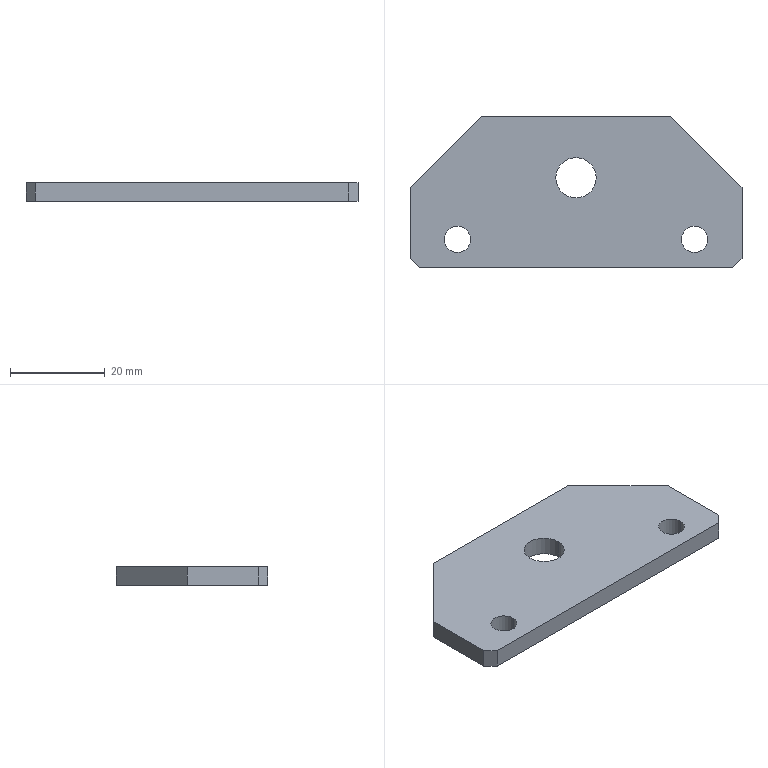Component | SolidWorks | DZ.KX.203-TC1505-30-09-01-05-03-4 | 1 solid | 16 faces | box 70 x 32 x 4 mm | volume 7627 mm3 | plane 10 | cylinder 6 | commonest cylinder face diameters 5.5 x4 8.5 x2
build123d program:
from build123d import *

# Parameters (mm, degrees)
SKETCH1_W                      = 70
SKETCH1_H                      = 32
BOSS_EXTRUDE1_DEPTH            = 4
HOLE1_D                        = 8.5
CHAMFER1_SIZE                  = 15
F_5_5_5_5_DIAMETER_HOLE1_D     = 5.5
F_5_5_5_5_DIAMETER_HOLE1_DEPTH = 5
CHAMFER2_SIZE                  = 2


with BuildPart() as part:
    # Sketch1 → Boss-Extrude1 (new body)
    with BuildSketch(Plane(origin=(0, 0, 0), x_dir=(0, 0, -1), z_dir=(1, 0, 0))):
        Rectangle(SKETCH1_W, SKETCH1_H)
    extrude(amount=BOSS_EXTRUDE1_DEPTH)

    # Hole1 (through all)
    with Locations(Plane.ZY):
        with Locations((0, -3)):
            Hole(HOLE1_D / 2)

    # Chamfer1
    chamfer1_edges = [part.edges().sort_by_distance(p)[0] for p in [
        (2, -16, -35),
        (2, -16, 35),
    ]]
    chamfer(chamfer1_edges, length=CHAMFER1_SIZE)

    # 5.5 _5.5_ Diameter Hole1
    with Locations(Plane.ZY):
        with Locations((-25, 10), (25, 10)):
            Hole(F_5_5_5_5_DIAMETER_HOLE1_D / 2, depth=F_5_5_5_5_DIAMETER_HOLE1_DEPTH)

    # Chamfer2
    chamfer2_edges = [part.edges().sort_by_distance(p)[0] for p in [
        (2, 16, 35),
        (2, 16, -35),
    ]]
    chamfer(chamfer2_edges, length=CHAMFER2_SIZE)


solid = part.part

# Placed as in the assembly
solid = solid.moved(Location((294.5, -579.307, 49.441), (180, 90, 0)))
STEP:
#1=COLOUR_RGB('',0.7922,0.8196,0.9333);
#2=FILL_AREA_STYLE_COLOUR('',#1);
#3=FILL_AREA_STYLE('',(#2));
#4=SURFACE_STYLE_FILL_AREA(#3);
#5=SURFACE_SIDE_STYLE('',(#4));
#6=SURFACE_STYLE_USAGE(.BOTH.,#5);
#7=PRESENTATION_STYLE_ASSIGNMENT((#6));
#8=CARTESIAN_POINT('',(10.719,-23.201,2.104));
#9=VERTEX_POINT('',#8);
#10=CARTESIAN_POINT('',(10.502,-23.201,2.104));
#11=VERTEX_POINT('',#10);
#12=CARTESIAN_POINT('',(10.61,-23.201,2.104));
#13=DIRECTION('',(0.,0.,1.));
#14=DIRECTION('',(-1.,0.,0.));
#15=AXIS2_PLACEMENT_3D('',#12,#13,#14);
#16=CIRCLE('',#15,0.1083);
#17=EDGE_CURVE('',#9,#11,#16,.T.);
#18=ORIENTED_EDGE('',*,*,#17,.T.);
#19=CARTESIAN_POINT('',(10.502,-23.201,1.946));
#20=VERTEX_POINT('',#19);
#21=CARTESIAN_POINT('',(10.502,-23.201,1.946));
#22=DIRECTION('',(-0.,-0.,-1.));
#23=VECTOR('',#22,39.37);
#24=LINE('',#21,#23);
#25=EDGE_CURVE('',#11,#20,#24,.T.);
#26=ORIENTED_EDGE('',*,*,#25,.T.);
#27=CARTESIAN_POINT('',(10.719,-23.201,1.946));
#28=VERTEX_POINT('',#27);
#29=CARTESIAN_POINT('',(10.61,-23.201,1.946));
#30=DIRECTION('',(-0.,-0.,-1.));
#31=DIRECTION('',(1.,0.,0.));
#32=AXIS2_PLACEMENT_3D('',#29,#30,#31);
#33=CIRCLE('',#32,0.1083);
#34=EDGE_CURVE('',#20,#28,#33,.T.);
#35=ORIENTED_EDGE('',*,*,#34,.T.);
#36=CARTESIAN_POINT('',(10.719,-23.201,1.946));
#37=DIRECTION('',(-0.,-0.,-1.));
#38=VECTOR('',#37,39.37);
#39=LINE('',#36,#38);
#40=EDGE_CURVE('',#9,#28,#39,.T.);
#41=ORIENTED_EDGE('',*,*,#40,.F.);
#42=EDGE_LOOP('',(#18,#26,#35,#41));
#43=FACE_OUTER_BOUND('',#42,.T.);
#44=CARTESIAN_POINT('',(10.61,-23.201,1.946));
#45=DIRECTION('',(-0.,-0.,-1.));
#46=DIRECTION('',(1.,0.,0.));
#47=AXIS2_PLACEMENT_3D('',#44,#45,#46);
#48=CYLINDRICAL_SURFACE('',#47,0.1083);
#49=ADVANCED_FACE('',(#43),#48,.F.);
#50=CARTESIAN_POINT('',(12.687,-23.201,2.104));
#51=VERTEX_POINT('',#50);
#52=CARTESIAN_POINT('',(12.47,-23.201,2.104));
#53=VERTEX_POINT('',#52);
#54=CARTESIAN_POINT('',(12.579,-23.201,2.104));
#55=DIRECTION('',(0.,0.,1.));
#56=DIRECTION('',(-1.,0.,0.));
#57=AXIS2_PLACEMENT_3D('',#54,#55,#56);
#58=CIRCLE('',#57,0.1083);
#59=EDGE_CURVE('',#51,#53,#58,.T.);
#60=ORIENTED_EDGE('',*,*,#59,.T.);
#61=CARTESIAN_POINT('',(12.47,-23.201,1.946));
#62=VERTEX_POINT('',#61);
#63=CARTESIAN_POINT('',(12.47,-23.201,1.946));
#64=DIRECTION('',(-0.,-0.,-1.));
#65=VECTOR('',#64,39.37);
#66=LINE('',#63,#65);
#67=EDGE_CURVE('',#53,#62,#66,.T.);
#68=ORIENTED_EDGE('',*,*,#67,.T.);
#69=CARTESIAN_POINT('',(12.687,-23.201,1.946));
#70=VERTEX_POINT('',#69);
#71=CARTESIAN_POINT('',(12.579,-23.201,1.946));
#72=DIRECTION('',(-0.,-0.,-1.));
#73=DIRECTION('',(1.,0.,0.));
#74=AXIS2_PLACEMENT_3D('',#71,#72,#73);
#75=CIRCLE('',#74,0.1083);
#76=EDGE_CURVE('',#62,#70,#75,.T.);
#77=ORIENTED_EDGE('',*,*,#76,.T.);
#78=CARTESIAN_POINT('',(12.687,-23.201,1.946));
#79=DIRECTION('',(-0.,-0.,-1.));
#80=VECTOR('',#79,39.37);
#81=LINE('',#78,#80);
#82=EDGE_CURVE('',#51,#70,#81,.T.);
#83=ORIENTED_EDGE('',*,*,#82,.F.);
#84=EDGE_LOOP('',(#60,#68,#77,#83));
#85=FACE_OUTER_BOUND('',#84,.T.);
#86=CARTESIAN_POINT('',(12.579,-23.201,1.946));
#87=DIRECTION('',(-0.,-0.,-1.));
#88=DIRECTION('',(1.,0.,0.));
#89=AXIS2_PLACEMENT_3D('',#86,#87,#88);
#90=CYLINDRICAL_SURFACE('',#89,0.1083);
#91=ADVANCED_FACE('',(#85),#90,.F.);
#92=CARTESIAN_POINT('',(11.427,-22.689,2.104));
#93=VERTEX_POINT('',#92);
#94=CARTESIAN_POINT('',(11.762,-22.689,2.104));
#95=VERTEX_POINT('',#94);
#96=CARTESIAN_POINT('',(11.594,-22.689,2.104));
#97=DIRECTION('',(-0.,-0.,-1.));
#98=DIRECTION('',(1.,0.,0.));
#99=AXIS2_PLACEMENT_3D('',#96,#97,#98);
#100=CIRCLE('',#99,0.1673);
#101=EDGE_CURVE('',#93,#95,#100,.T.);
#102=ORIENTED_EDGE('',*,*,#101,.F.);
#103=CARTESIAN_POINT('',(11.427,-22.689,1.946));
#104=VERTEX_POINT('',#103);
#105=CARTESIAN_POINT('',(11.427,-22.689,1.946));
#106=DIRECTION('',(-0.,-0.,-1.));
#107=VECTOR('',#106,39.37);
#108=LINE('',#105,#107);
#109=EDGE_CURVE('',#93,#104,#108,.T.);
#110=ORIENTED_EDGE('',*,*,#109,.T.);
#111=CARTESIAN_POINT('',(11.762,-22.689,1.946));
#112=VERTEX_POINT('',#111);
#113=CARTESIAN_POINT('',(11.594,-22.689,1.946));
#114=DIRECTION('',(-0.,-0.,-1.));
#115=DIRECTION('',(1.,0.,0.));
#116=AXIS2_PLACEMENT_3D('',#113,#114,#115);
#117=CIRCLE('',#116,0.1673);
#118=EDGE_CURVE('',#104,#112,#117,.T.);
#119=ORIENTED_EDGE('',*,*,#118,.T.);
#120=CARTESIAN_POINT('',(11.762,-22.689,1.946));
#121=DIRECTION('',(-0.,-0.,-1.));
#122=VECTOR('',#121,39.37);
#123=LINE('',#120,#122);
#124=EDGE_CURVE('',#95,#112,#123,.T.);
#125=ORIENTED_EDGE('',*,*,#124,.F.);
#126=EDGE_LOOP('',(#102,#110,#119,#125));
#127=FACE_OUTER_BOUND('',#126,.T.);
#128=CARTESIAN_POINT('',(11.594,-22.689,1.946));
#129=DIRECTION('',(-0.,-0.,-1.));
#130=DIRECTION('',(1.,0.,0.));
#131=AXIS2_PLACEMENT_3D('',#128,#129,#130);
#132=CYLINDRICAL_SURFACE('',#131,0.1673);
#133=ADVANCED_FACE('',(#127),#132,.F.);
#134=CARTESIAN_POINT('',(12.972,-23.359,2.104));
#135=VERTEX_POINT('',#134);
#136=CARTESIAN_POINT('',(12.972,-22.768,2.104));
#137=VERTEX_POINT('',#136);
#138=CARTESIAN_POINT('',(12.972,-22.177,2.104));
#139=DIRECTION('',(0.,1.,-0.));
#140=VECTOR('',#139,39.37);
#141=LINE('',#138,#140);
#142=EDGE_CURVE('',#135,#137,#141,.T.);
#143=ORIENTED_EDGE('',*,*,#142,.F.);
#144=CARTESIAN_POINT('',(12.972,-23.359,1.946));
#145=VERTEX_POINT('',#144);
#146=CARTESIAN_POINT('',(12.972,-23.359,2.104));
#147=DIRECTION('',(-0.,-0.,-1.));
#148=VECTOR('',#147,39.37);
#149=LINE('',#146,#148);
#150=EDGE_CURVE('',#135,#145,#149,.T.);
#151=ORIENTED_EDGE('',*,*,#150,.T.);
#152=CARTESIAN_POINT('',(12.972,-22.768,1.946));
#153=VERTEX_POINT('',#152);
#154=CARTESIAN_POINT('',(12.972,-22.177,1.946));
#155=DIRECTION('',(0.,1.,-0.));
#156=VECTOR('',#155,39.37);
#157=LINE('',#154,#156);
#158=EDGE_CURVE('',#145,#153,#157,.T.);
#159=ORIENTED_EDGE('',*,*,#158,.T.);
#160=CARTESIAN_POINT('',(12.972,-22.768,2.104));
#161=DIRECTION('',(0.,0.,1.));
#162=VECTOR('',#161,39.37);
#163=LINE('',#160,#162);
#164=EDGE_CURVE('',#153,#137,#163,.T.);
#165=ORIENTED_EDGE('',*,*,#164,.T.);
#166=EDGE_LOOP('',(#143,#151,#159,#165));
#167=FACE_OUTER_BOUND('',#166,.T.);
#168=CARTESIAN_POINT('',(12.972,-22.177,2.104));
#169=DIRECTION('',(-1.,0.,0.));
#170=DIRECTION('',(-0.,-0.,-1.));
#171=AXIS2_PLACEMENT_3D('',#168,#169,#170);
#172=PLANE('',#171);
#173=ADVANCED_FACE('',(#167),#172,.F.);
#174=CARTESIAN_POINT('',(12.382,-22.177,2.104));
#175=VERTEX_POINT('',#174);
#176=CARTESIAN_POINT('',(10.807,-22.177,2.104));
#177=VERTEX_POINT('',#176);
#178=CARTESIAN_POINT('',(10.217,-22.177,2.104));
#179=DIRECTION('',(-1.,0.,0.));
#180=VECTOR('',#179,39.37);
#181=LINE('',#178,#180);
#182=EDGE_CURVE('',#175,#177,#181,.T.);
#183=ORIENTED_EDGE('',*,*,#182,.F.);
#184=CARTESIAN_POINT('',(12.382,-22.177,1.946));
#185=VERTEX_POINT('',#184);
#186=CARTESIAN_POINT('',(12.382,-22.177,2.104));
#187=DIRECTION('',(-0.,-0.,-1.));
#188=VECTOR('',#187,39.37);
#189=LINE('',#186,#188);
#190=EDGE_CURVE('',#175,#185,#189,.T.);
#191=ORIENTED_EDGE('',*,*,#190,.T.);
#192=CARTESIAN_POINT('',(10.807,-22.177,1.946));
#193=VERTEX_POINT('',#192);
#194=CARTESIAN_POINT('',(10.217,-22.177,1.946));
#195=DIRECTION('',(-1.,0.,0.));
#196=VECTOR('',#195,39.37);
#197=LINE('',#194,#196);
#198=EDGE_CURVE('',#185,#193,#197,.T.);
#199=ORIENTED_EDGE('',*,*,#198,.T.);
#200=CARTESIAN_POINT('',(10.807,-22.177,2.104));
#201=DIRECTION('',(0.,0.,1.));
#202=VECTOR('',#201,39.37);
#203=LINE('',#200,#202);
#204=EDGE_CURVE('',#193,#177,#203,.T.);
#205=ORIENTED_EDGE('',*,*,#204,.T.);
#206=EDGE_LOOP('',(#183,#191,#199,#205));
#207=FACE_OUTER_BOUND('',#206,.T.);
#208=CARTESIAN_POINT('',(10.217,-22.177,2.104));
#209=DIRECTION('',(-0.,-1.,0.));
#210=DIRECTION('',(1.,-0.,-0.));
#211=AXIS2_PLACEMENT_3D('',#208,#209,#210);
#212=PLANE('',#211);
#213=ADVANCED_FACE('',(#207),#212,.F.);
#214=CARTESIAN_POINT('',(10.217,-22.768,1.946));
#215=VERTEX_POINT('',#214);
#216=CARTESIAN_POINT('',(10.217,-23.359,1.946));
#217=VERTEX_POINT('',#216);
#218=CARTESIAN_POINT('',(10.217,-22.177,1.946));
#219=DIRECTION('',(-0.,-1.,0.));
#220=VECTOR('',#219,39.37);
#221=LINE('',#218,#220);
#222=EDGE_CURVE('',#215,#217,#221,.T.);
#223=ORIENTED_EDGE('',*,*,#222,.T.);
#224=CARTESIAN_POINT('',(10.217,-23.359,2.104));
#225=VERTEX_POINT('',#224);
#226=CARTESIAN_POINT('',(10.217,-23.359,2.104));
#227=DIRECTION('',(0.,0.,1.));
#228=VECTOR('',#227,39.37);
#229=LINE('',#226,#228);
#230=EDGE_CURVE('',#217,#225,#229,.T.);
#231=ORIENTED_EDGE('',*,*,#230,.T.);
#232=CARTESIAN_POINT('',(10.217,-22.768,2.104));
#233=VERTEX_POINT('',#232);
#234=CARTESIAN_POINT('',(10.217,-22.177,2.104));
#235=DIRECTION('',(-0.,-1.,0.));
#236=VECTOR('',#235,39.37);
#237=LINE('',#234,#236);
#238=EDGE_CURVE('',#233,#225,#237,.T.);
#239=ORIENTED_EDGE('',*,*,#238,.F.);
#240=CARTESIAN_POINT('',(10.217,-22.768,2.104));
#241=DIRECTION('',(-0.,-0.,-1.));
#242=VECTOR('',#241,39.37);
#243=LINE('',#240,#242);
#244=EDGE_CURVE('',#233,#215,#243,.T.);
#245=ORIENTED_EDGE('',*,*,#244,.T.);
#246=EDGE_LOOP('',(#223,#231,#239,#245));
#247=FACE_OUTER_BOUND('',#246,.T.);
#248=CARTESIAN_POINT('',(10.217,-22.177,2.104));
#249=DIRECTION('',(1.,-0.,-0.));
#250=DIRECTION('',(0.,0.,1.));
#251=AXIS2_PLACEMENT_3D('',#248,#249,#250);
#252=PLANE('',#251);
#253=ADVANCED_FACE('',(#247),#252,.F.);
#254=CARTESIAN_POINT('',(10.295,-23.437,2.104));
#255=VERTEX_POINT('',#254);
#256=CARTESIAN_POINT('',(12.894,-23.437,2.104));
#257=VERTEX_POINT('',#256);
#258=CARTESIAN_POINT('',(10.217,-23.437,2.104));
#259=DIRECTION('',(1.,-0.,-0.));
#260=VECTOR('',#259,39.37);
#261=LINE('',#258,#260);
#262=EDGE_CURVE('',#255,#257,#261,.T.);
#263=ORIENTED_EDGE('',*,*,#262,.F.);
#264=CARTESIAN_POINT('',(10.295,-23.437,1.946));
#265=VERTEX_POINT('',#264);
#266=CARTESIAN_POINT('',(10.295,-23.437,2.104));
#267=DIRECTION('',(-0.,-0.,-1.));
#268=VECTOR('',#267,39.37);
#269=LINE('',#266,#268);
#270=EDGE_CURVE('',#255,#265,#269,.T.);
#271=ORIENTED_EDGE('',*,*,#270,.T.);
#272=CARTESIAN_POINT('',(12.894,-23.437,1.946));
#273=VERTEX_POINT('',#272);
#274=CARTESIAN_POINT('',(10.217,-23.437,1.946));
#275=DIRECTION('',(1.,-0.,-0.));
#276=VECTOR('',#275,39.37);
#277=LINE('',#274,#276);
#278=EDGE_CURVE('',#265,#273,#277,.T.);
#279=ORIENTED_EDGE('',*,*,#278,.T.);
#280=CARTESIAN_POINT('',(12.894,-23.437,2.104));
#281=DIRECTION('',(0.,0.,1.));
#282=VECTOR('',#281,39.37);
#283=LINE('',#280,#282);
#284=EDGE_CURVE('',#273,#257,#283,.T.);
#285=ORIENTED_EDGE('',*,*,#284,.T.);
#286=EDGE_LOOP('',(#263,#271,#279,#285));
#287=FACE_OUTER_BOUND('',#286,.T.);
#288=CARTESIAN_POINT('',(10.217,-23.437,2.104));
#289=DIRECTION('',(0.,1.,-0.));
#290=DIRECTION('',(-1.,0.,0.));
#291=AXIS2_PLACEMENT_3D('',#288,#289,#290);
#292=PLANE('',#291);
#293=ADVANCED_FACE('',(#287),#292,.F.);
#294=ORIENTED_EDGE('',*,*,#17,.F.);
#295=CARTESIAN_POINT('',(10.61,-23.201,2.104));
#296=DIRECTION('',(0.,0.,1.));
#297=DIRECTION('',(-1.,0.,0.));
#298=AXIS2_PLACEMENT_3D('',#295,#296,#297);
#299=CIRCLE('',#298,0.1083);
#300=EDGE_CURVE('',#11,#9,#299,.T.);
#301=ORIENTED_EDGE('',*,*,#300,.F.);
#302=EDGE_LOOP('',(#294,#301));
#303=FACE_BOUND('',#302,.T.);
#304=ORIENTED_EDGE('',*,*,#59,.F.);
#305=CARTESIAN_POINT('',(12.579,-23.201,2.104));
#306=DIRECTION('',(0.,0.,1.));
#307=DIRECTION('',(-1.,0.,0.));
#308=AXIS2_PLACEMENT_3D('',#305,#306,#307);
#309=CIRCLE('',#308,0.1083);
#310=EDGE_CURVE('',#53,#51,#309,.T.);
#311=ORIENTED_EDGE('',*,*,#310,.F.);
#312=EDGE_LOOP('',(#304,#311));
#313=FACE_BOUND('',#312,.T.);
#314=CARTESIAN_POINT('',(11.594,-22.689,2.104));
#315=DIRECTION('',(-0.,-0.,-1.));
#316=DIRECTION('',(1.,0.,0.));
#317=AXIS2_PLACEMENT_3D('',#314,#315,#316);
#318=CIRCLE('',#317,0.1673);
#319=EDGE_CURVE('',#95,#93,#318,.T.);
#320=ORIENTED_EDGE('',*,*,#319,.T.);
#321=ORIENTED_EDGE('',*,*,#101,.T.);
#322=EDGE_LOOP('',(#320,#321));
#323=FACE_BOUND('',#322,.T.);
#324=ORIENTED_EDGE('',*,*,#238,.T.);
#325=CARTESIAN_POINT('',(10.63,-23.772,2.104));
#326=DIRECTION('',(0.7071,-0.7071,0.));
#327=VECTOR('',#326,39.37);
#328=LINE('',#325,#327);
#329=EDGE_CURVE('',#225,#255,#328,.T.);
#330=ORIENTED_EDGE('',*,*,#329,.T.);
#331=ORIENTED_EDGE('',*,*,#262,.T.);
#332=CARTESIAN_POINT('',(12.559,-23.772,2.104));
#333=DIRECTION('',(0.7071,0.7071,-0.));
#334=VECTOR('',#333,39.37);
#335=LINE('',#332,#334);
#336=EDGE_CURVE('',#257,#135,#335,.T.);
#337=ORIENTED_EDGE('',*,*,#336,.T.);
#338=ORIENTED_EDGE('',*,*,#142,.T.);
#339=CARTESIAN_POINT('',(12.303,-22.099,2.104));
#340=DIRECTION('',(-0.7071,0.7071,-0.));
#341=VECTOR('',#340,39.37);
#342=LINE('',#339,#341);
#343=EDGE_CURVE('',#137,#175,#342,.T.);
#344=ORIENTED_EDGE('',*,*,#343,.T.);
#345=ORIENTED_EDGE('',*,*,#182,.T.);
#346=CARTESIAN_POINT('',(10.886,-22.099,2.104));
#347=DIRECTION('',(-0.7071,-0.7071,0.));
#348=VECTOR('',#347,39.37);
#349=LINE('',#346,#348);
#350=EDGE_CURVE('',#177,#233,#349,.T.);
#351=ORIENTED_EDGE('',*,*,#350,.T.);
#352=EDGE_LOOP('',(#324,#330,#331,#337,#338,#344,#345,#351));
#353=FACE_OUTER_BOUND('',#352,.T.);
#354=CARTESIAN_POINT('',(11.594,-22.807,2.104));
#355=DIRECTION('',(0.,0.,1.));
#356=DIRECTION('',(-1.,0.,0.));
#357=AXIS2_PLACEMENT_3D('',#354,#355,#356);
#358=PLANE('',#357);
#359=ADVANCED_FACE('',(#303,#313,#323,#353),#358,.T.);
#360=CARTESIAN_POINT('',(10.61,-23.201,1.946));
#361=DIRECTION('',(-0.,-0.,-1.));
#362=DIRECTION('',(1.,0.,0.));
#363=AXIS2_PLACEMENT_3D('',#360,#361,#362);
#364=CIRCLE('',#363,0.1083);
#365=EDGE_CURVE('',#28,#20,#364,.T.);
#366=ORIENTED_EDGE('',*,*,#365,.F.);
#367=ORIENTED_EDGE('',*,*,#34,.F.);
#368=EDGE_LOOP('',(#366,#367));
#369=FACE_BOUND('',#368,.T.);
#370=CARTESIAN_POINT('',(12.579,-23.201,1.946));
#371=DIRECTION('',(-0.,-0.,-1.));
#372=DIRECTION('',(1.,0.,0.));
#373=AXIS2_PLACEMENT_3D('',#370,#371,#372);
#374=CIRCLE('',#373,0.1083);
#375=EDGE_CURVE('',#70,#62,#374,.T.);
#376=ORIENTED_EDGE('',*,*,#375,.F.);
#377=ORIENTED_EDGE('',*,*,#76,.F.);
#378=EDGE_LOOP('',(#376,#377));
#379=FACE_BOUND('',#378,.T.);
#380=CARTESIAN_POINT('',(11.594,-22.689,1.946));
#381=DIRECTION('',(-0.,-0.,-1.));
#382=DIRECTION('',(1.,0.,0.));
#383=AXIS2_PLACEMENT_3D('',#380,#381,#382);
#384=CIRCLE('',#383,0.1673);
#385=EDGE_CURVE('',#112,#104,#384,.T.);
#386=ORIENTED_EDGE('',*,*,#385,.F.);
#387=ORIENTED_EDGE('',*,*,#118,.F.);
#388=EDGE_LOOP('',(#386,#387));
#389=FACE_BOUND('',#388,.T.);
#390=ORIENTED_EDGE('',*,*,#278,.F.);
#391=CARTESIAN_POINT('',(10.295,-23.437,1.946));
#392=DIRECTION('',(-0.7071,0.7071,-0.));
#393=VECTOR('',#392,39.37);
#394=LINE('',#391,#393);
#395=EDGE_CURVE('',#265,#217,#394,.T.);
#396=ORIENTED_EDGE('',*,*,#395,.T.);
#397=ORIENTED_EDGE('',*,*,#222,.F.);
#398=CARTESIAN_POINT('',(10.217,-22.768,1.946));
#399=DIRECTION('',(0.7071,0.7071,-0.));
#400=VECTOR('',#399,39.37);
#401=LINE('',#398,#400);
#402=EDGE_CURVE('',#215,#193,#401,.T.);
#403=ORIENTED_EDGE('',*,*,#402,.T.);
#404=ORIENTED_EDGE('',*,*,#198,.F.);
#405=CARTESIAN_POINT('',(12.382,-22.177,1.946));
#406=DIRECTION('',(0.7071,-0.7071,0.));
#407=VECTOR('',#406,39.37);
#408=LINE('',#405,#407);
#409=EDGE_CURVE('',#185,#153,#408,.T.);
#410=ORIENTED_EDGE('',*,*,#409,.T.);
#411=ORIENTED_EDGE('',*,*,#158,.F.);
#412=CARTESIAN_POINT('',(12.972,-23.359,1.946));
#413=DIRECTION('',(-0.7071,-0.7071,0.));
#414=VECTOR('',#413,39.37);
#415=LINE('',#412,#414);
#416=EDGE_CURVE('',#145,#273,#415,.T.);
#417=ORIENTED_EDGE('',*,*,#416,.T.);
#418=EDGE_LOOP('',(#390,#396,#397,#403,#404,#410,#411,#417));
#419=FACE_OUTER_BOUND('',#418,.T.);
#420=CARTESIAN_POINT('',(11.594,-22.807,1.946));
#421=DIRECTION('',(0.,0.,1.));
#422=DIRECTION('',(-1.,0.,0.));
#423=AXIS2_PLACEMENT_3D('',#420,#421,#422);
#424=PLANE('',#423);
#425=ADVANCED_FACE('',(#369,#379,#389,#419),#424,.F.);
#426=ORIENTED_EDGE('',*,*,#109,.F.);
#427=ORIENTED_EDGE('',*,*,#319,.F.);
#428=ORIENTED_EDGE('',*,*,#124,.T.);
#429=ORIENTED_EDGE('',*,*,#385,.T.);
#430=EDGE_LOOP('',(#426,#427,#428,#429));
#431=FACE_OUTER_BOUND('',#430,.T.);
#432=CARTESIAN_POINT('',(11.594,-22.689,1.946));
#433=DIRECTION('',(-0.,-0.,-1.));
#434=DIRECTION('',(1.,0.,0.));
#435=AXIS2_PLACEMENT_3D('',#432,#433,#434);
#436=CYLINDRICAL_SURFACE('',#435,0.1673);
#437=ADVANCED_FACE('',(#431),#436,.F.);
#438=ORIENTED_EDGE('',*,*,#343,.F.);
#439=ORIENTED_EDGE('',*,*,#164,.F.);
#440=ORIENTED_EDGE('',*,*,#409,.F.);
#441=ORIENTED_EDGE('',*,*,#190,.F.);
#442=EDGE_LOOP('',(#438,#439,#440,#441));
#443=FACE_OUTER_BOUND('',#442,.T.);
#444=CARTESIAN_POINT('',(12.382,-22.177,2.104));
#445=DIRECTION('',(-0.7071,-0.7071,0.));
#446=DIRECTION('',(-0.,-0.,-1.));
#447=AXIS2_PLACEMENT_3D('',#444,#445,#446);
#448=PLANE('',#447);
#449=ADVANCED_FACE('',(#443),#448,.F.);
#450=ORIENTED_EDGE('',*,*,#350,.F.);
#451=ORIENTED_EDGE('',*,*,#204,.F.);
#452=ORIENTED_EDGE('',*,*,#402,.F.);
#453=ORIENTED_EDGE('',*,*,#244,.F.);
#454=EDGE_LOOP('',(#450,#451,#452,#453));
#455=FACE_OUTER_BOUND('',#454,.T.);
#456=CARTESIAN_POINT('',(10.217,-22.768,2.104));
#457=DIRECTION('',(0.7071,-0.7071,0.));
#458=DIRECTION('',(-0.,-0.,-1.));
#459=AXIS2_PLACEMENT_3D('',#456,#457,#458);
#460=PLANE('',#459);
#461=ADVANCED_FACE('',(#455),#460,.F.);
#462=ORIENTED_EDGE('',*,*,#67,.F.);
#463=ORIENTED_EDGE('',*,*,#310,.T.);
#464=ORIENTED_EDGE('',*,*,#82,.T.);
#465=ORIENTED_EDGE('',*,*,#375,.T.);
#466=EDGE_LOOP('',(#462,#463,#464,#465));
#467=FACE_OUTER_BOUND('',#466,.T.);
#468=CARTESIAN_POINT('',(12.579,-23.201,1.946));
#469=DIRECTION('',(-0.,-0.,-1.));
#470=DIRECTION('',(1.,0.,0.));
#471=AXIS2_PLACEMENT_3D('',#468,#469,#470);
#472=CYLINDRICAL_SURFACE('',#471,0.1083);
#473=ADVANCED_FACE('',(#467),#472,.F.);
#474=ORIENTED_EDGE('',*,*,#25,.F.);
#475=ORIENTED_EDGE('',*,*,#300,.T.);
#476=ORIENTED_EDGE('',*,*,#40,.T.);
#477=ORIENTED_EDGE('',*,*,#365,.T.);
#478=EDGE_LOOP('',(#474,#475,#476,#477));
#479=FACE_OUTER_BOUND('',#478,.T.);
#480=CARTESIAN_POINT('',(10.61,-23.201,1.946));
#481=DIRECTION('',(-0.,-0.,-1.));
#482=DIRECTION('',(1.,0.,0.));
#483=AXIS2_PLACEMENT_3D('',#480,#481,#482);
#484=CYLINDRICAL_SURFACE('',#483,0.1083);
#485=ADVANCED_FACE('',(#479),#484,.F.);
#486=ORIENTED_EDGE('',*,*,#329,.F.);
#487=ORIENTED_EDGE('',*,*,#230,.F.);
#488=ORIENTED_EDGE('',*,*,#395,.F.);
#489=ORIENTED_EDGE('',*,*,#270,.F.);
#490=EDGE_LOOP('',(#486,#487,#488,#489));
#491=FACE_OUTER_BOUND('',#490,.T.);
#492=CARTESIAN_POINT('',(10.295,-23.437,2.104));
#493=DIRECTION('',(0.7071,0.7071,-0.));
#494=DIRECTION('',(-0.,-0.,-1.));
#495=AXIS2_PLACEMENT_3D('',#492,#493,#494);
#496=PLANE('',#495);
#497=ADVANCED_FACE('',(#491),#496,.F.);
#498=ORIENTED_EDGE('',*,*,#336,.F.);
#499=ORIENTED_EDGE('',*,*,#284,.F.);
#500=ORIENTED_EDGE('',*,*,#416,.F.);
#501=ORIENTED_EDGE('',*,*,#150,.F.);
#502=EDGE_LOOP('',(#498,#499,#500,#501));
#503=FACE_OUTER_BOUND('',#502,.T.);
#504=CARTESIAN_POINT('',(12.972,-23.359,2.104));
#505=DIRECTION('',(-0.7071,0.7071,-0.));
#506=DIRECTION('',(-0.,-0.,-1.));
#507=AXIS2_PLACEMENT_3D('',#504,#505,#506);
#508=PLANE('',#507);
#509=ADVANCED_FACE('',(#503),#508,.F.);
#510=CLOSED_SHELL('',(#49,#91,#133,#173,#213,#253,#293,#359,#425,#437,#449,#461,#473,#485,#497,#509));
#511=MANIFOLD_SOLID_BREP('',#510);
#512=STYLED_ITEM('',(#7),#511);
#513=(LENGTH_UNIT()NAMED_UNIT(*)SI_UNIT($,.METRE.));
#514=LENGTH_MEASURE_WITH_UNIT(LENGTH_MEASURE(0.0254),#513);
#515=DIMENSIONAL_EXPONENTS(1.,0.,0.,0.,0.,0.,0.);
#516=(CONVERSION_BASED_UNIT('',#514)LENGTH_UNIT()NAMED_UNIT(#515));
#517=UNCERTAINTY_MEASURE_WITH_UNIT(LENGTH_MEASURE(0.00001),#516,'','');
#518=(NAMED_UNIT(*)PLANE_ANGLE_UNIT()SI_UNIT($,.RADIAN.));
#519=(NAMED_UNIT(*)SI_UNIT($,.STERADIAN.)SOLID_ANGLE_UNIT());
#520=(GEOMETRIC_REPRESENTATION_CONTEXT(3)GLOBAL_UNCERTAINTY_ASSIGNED_CONTEXT((#517))GLOBAL_UNIT_ASSIGNED_CONTEXT((#516,#518,#519))REPRESENTATION_CONTEXT('',''));
#521=MECHANICAL_DESIGN_GEOMETRIC_PRESENTATION_REPRESENTATION('',(#512),#520);
#522=CARTESIAN_POINT('',(0.,0.,0.));
#523=DIRECTION('',(0.,0.,1.));
#524=DIRECTION('',(1.,0.,0.));
#525=AXIS2_PLACEMENT_3D('',#522,#523,#524);
#526=(LENGTH_UNIT()NAMED_UNIT(*)SI_UNIT($,.METRE.));
#527=LENGTH_MEASURE_WITH_UNIT(LENGTH_MEASURE(0.0254),#526);
#528=DIMENSIONAL_EXPONENTS(1.,0.,0.,0.,0.,0.,0.);
#529=(CONVERSION_BASED_UNIT('',#527)LENGTH_UNIT()NAMED_UNIT(#528));
#530=UNCERTAINTY_MEASURE_WITH_UNIT(LENGTH_MEASURE(0.00001),#529,'','');
#531=(NAMED_UNIT(*)PLANE_ANGLE_UNIT()SI_UNIT($,.RADIAN.));
#532=(NAMED_UNIT(*)SI_UNIT($,.STERADIAN.)SOLID_ANGLE_UNIT());
#533=(GEOMETRIC_REPRESENTATION_CONTEXT(3)GLOBAL_UNCERTAINTY_ASSIGNED_CONTEXT((#530))GLOBAL_UNIT_ASSIGNED_CONTEXT((#529,#531,#532))REPRESENTATION_CONTEXT('',''));
#534=ADVANCED_BREP_SHAPE_REPRESENTATION('',(#511,#525),#533);
#535=PRESENTATION_LAYER_ASSIGNMENT('','',(#512));